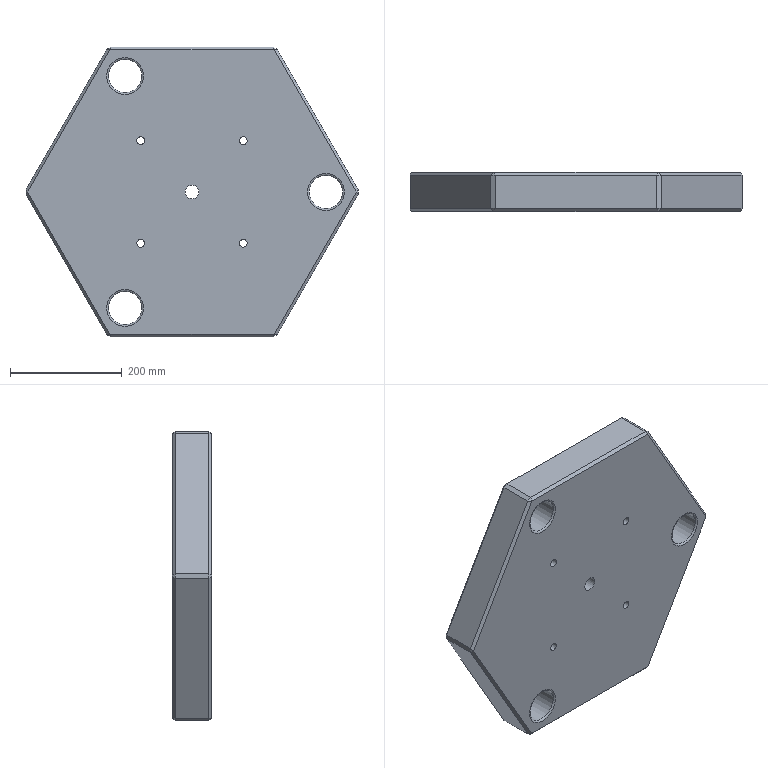Component | NX | TOP_PLATE | 1 solid | 76 faces | volume 15615563 mm3 | plane 42 | cylinder 16 | torus 10 | cone 8 | commonest cylinder face diameters 10 x4 14.2 x4 25.9 x4 60 x3 25 x1